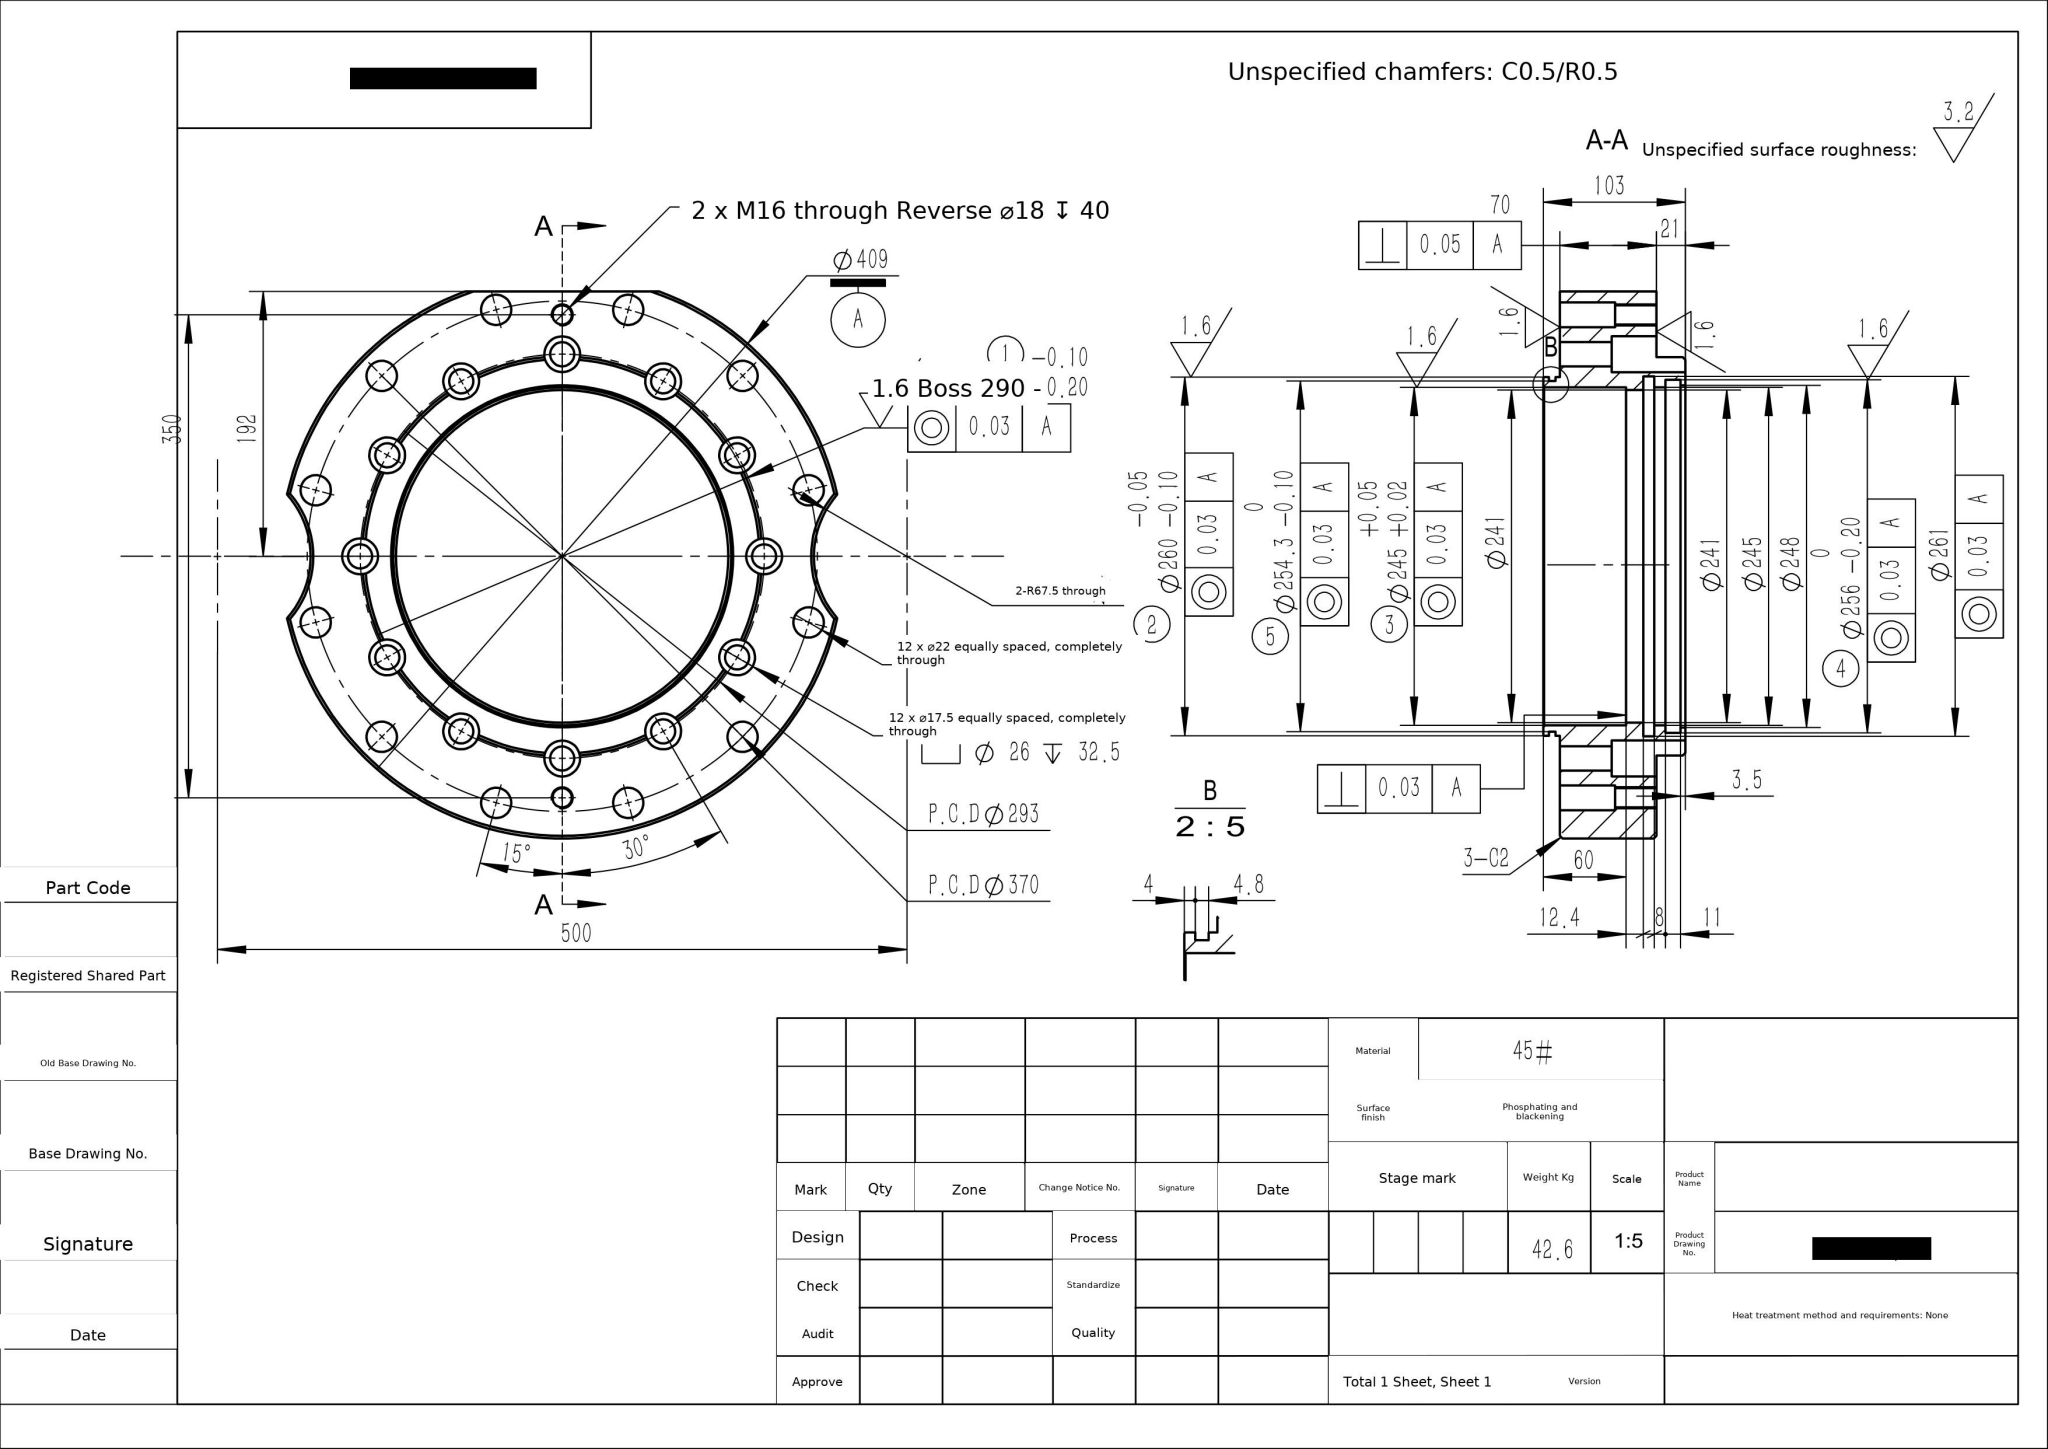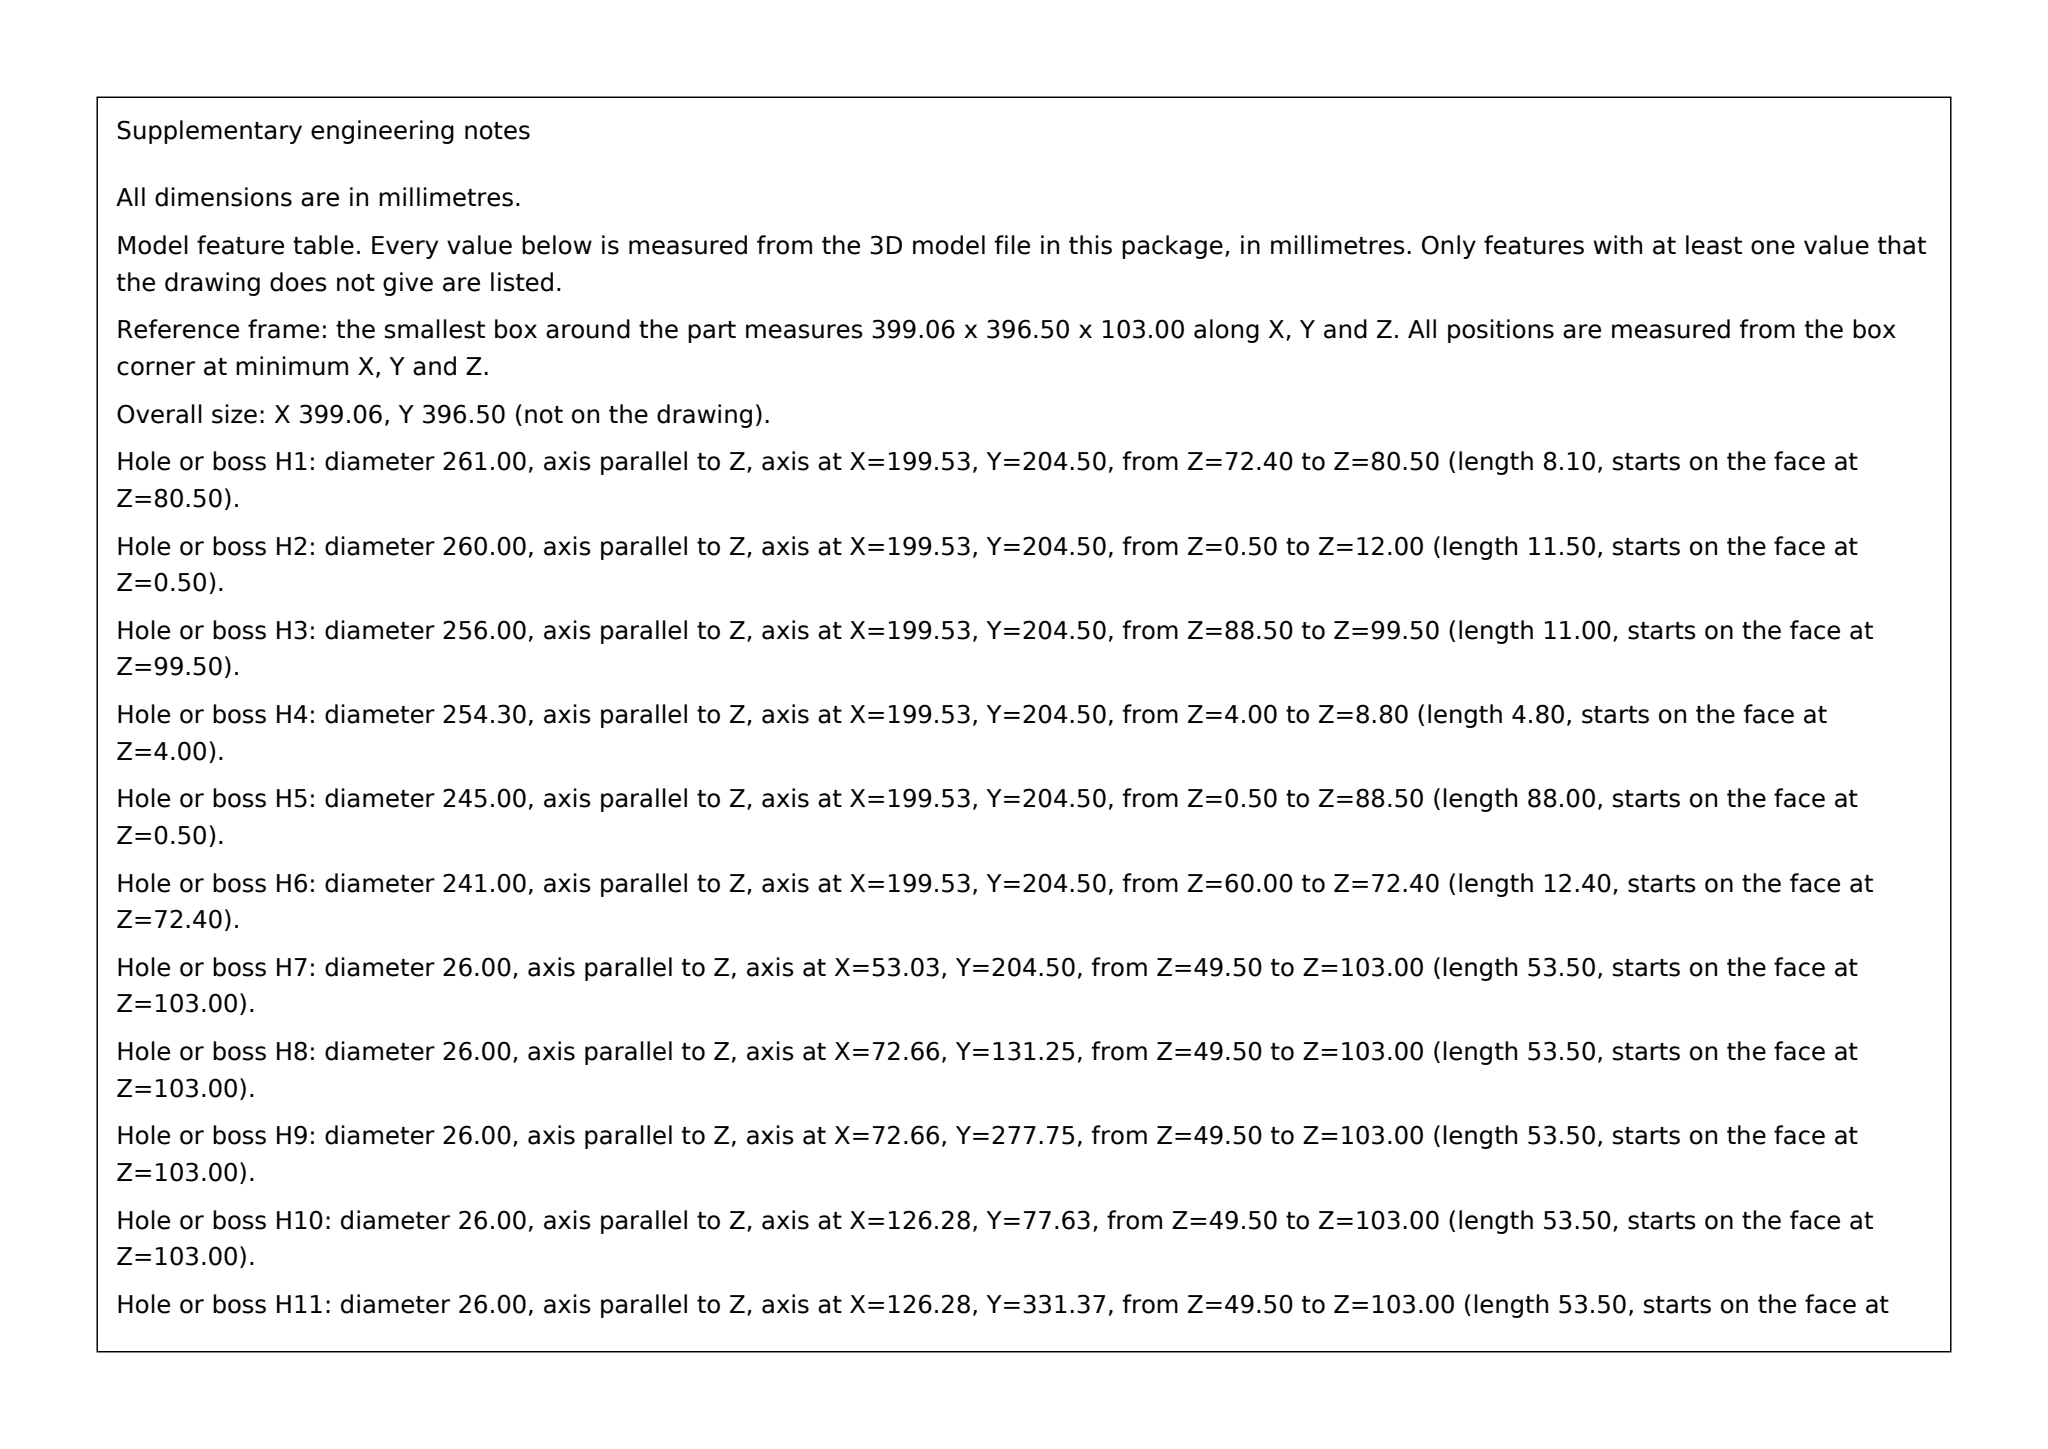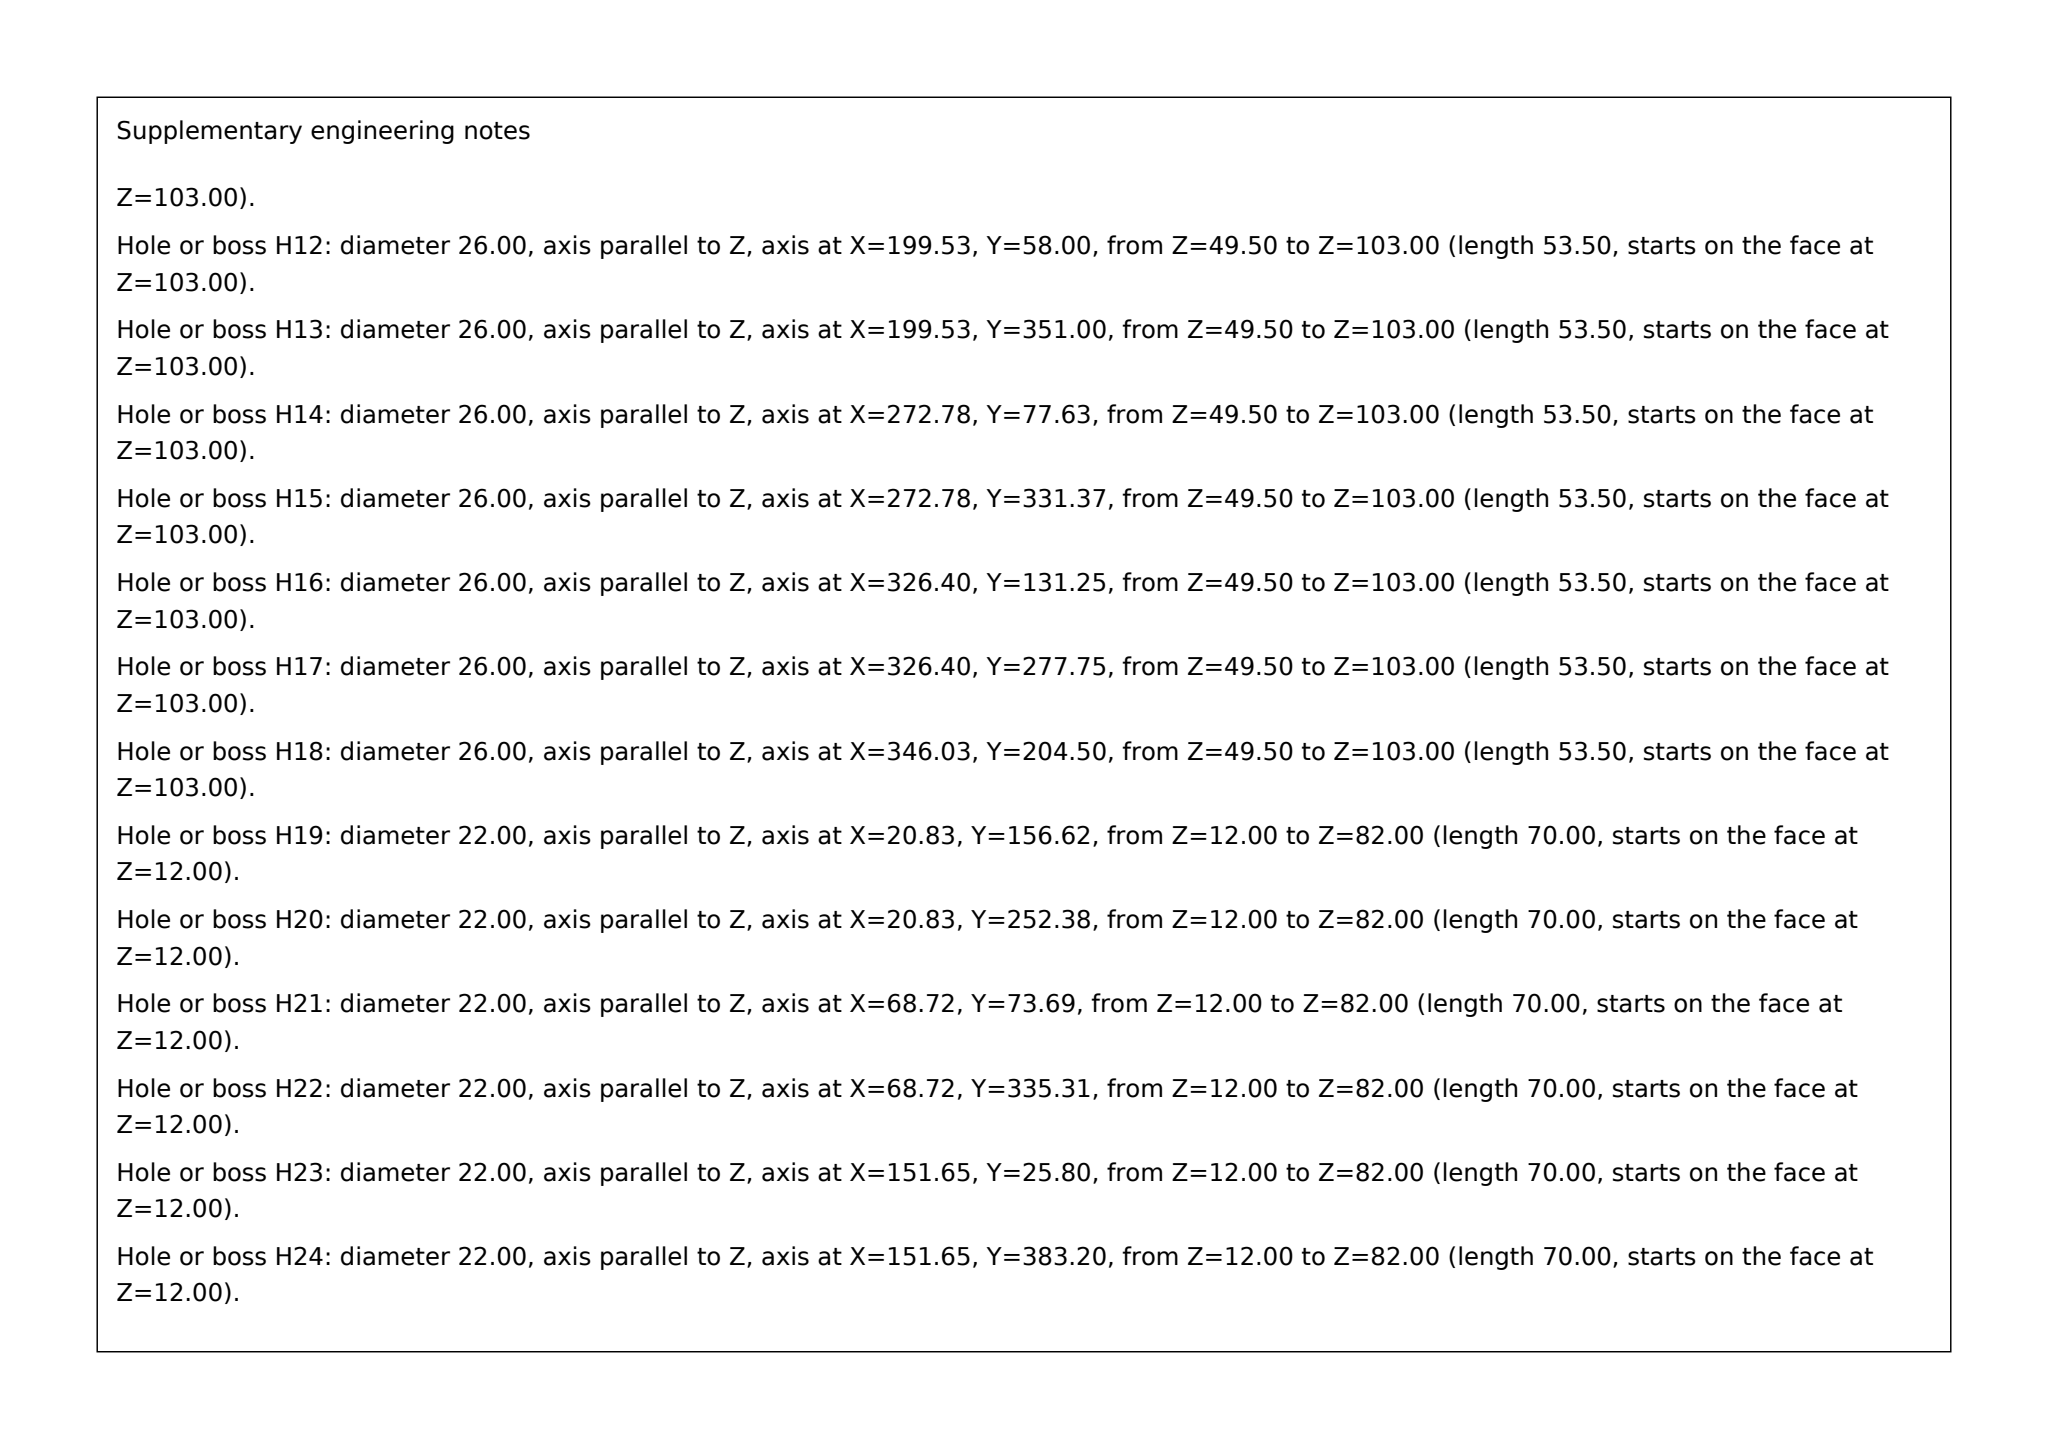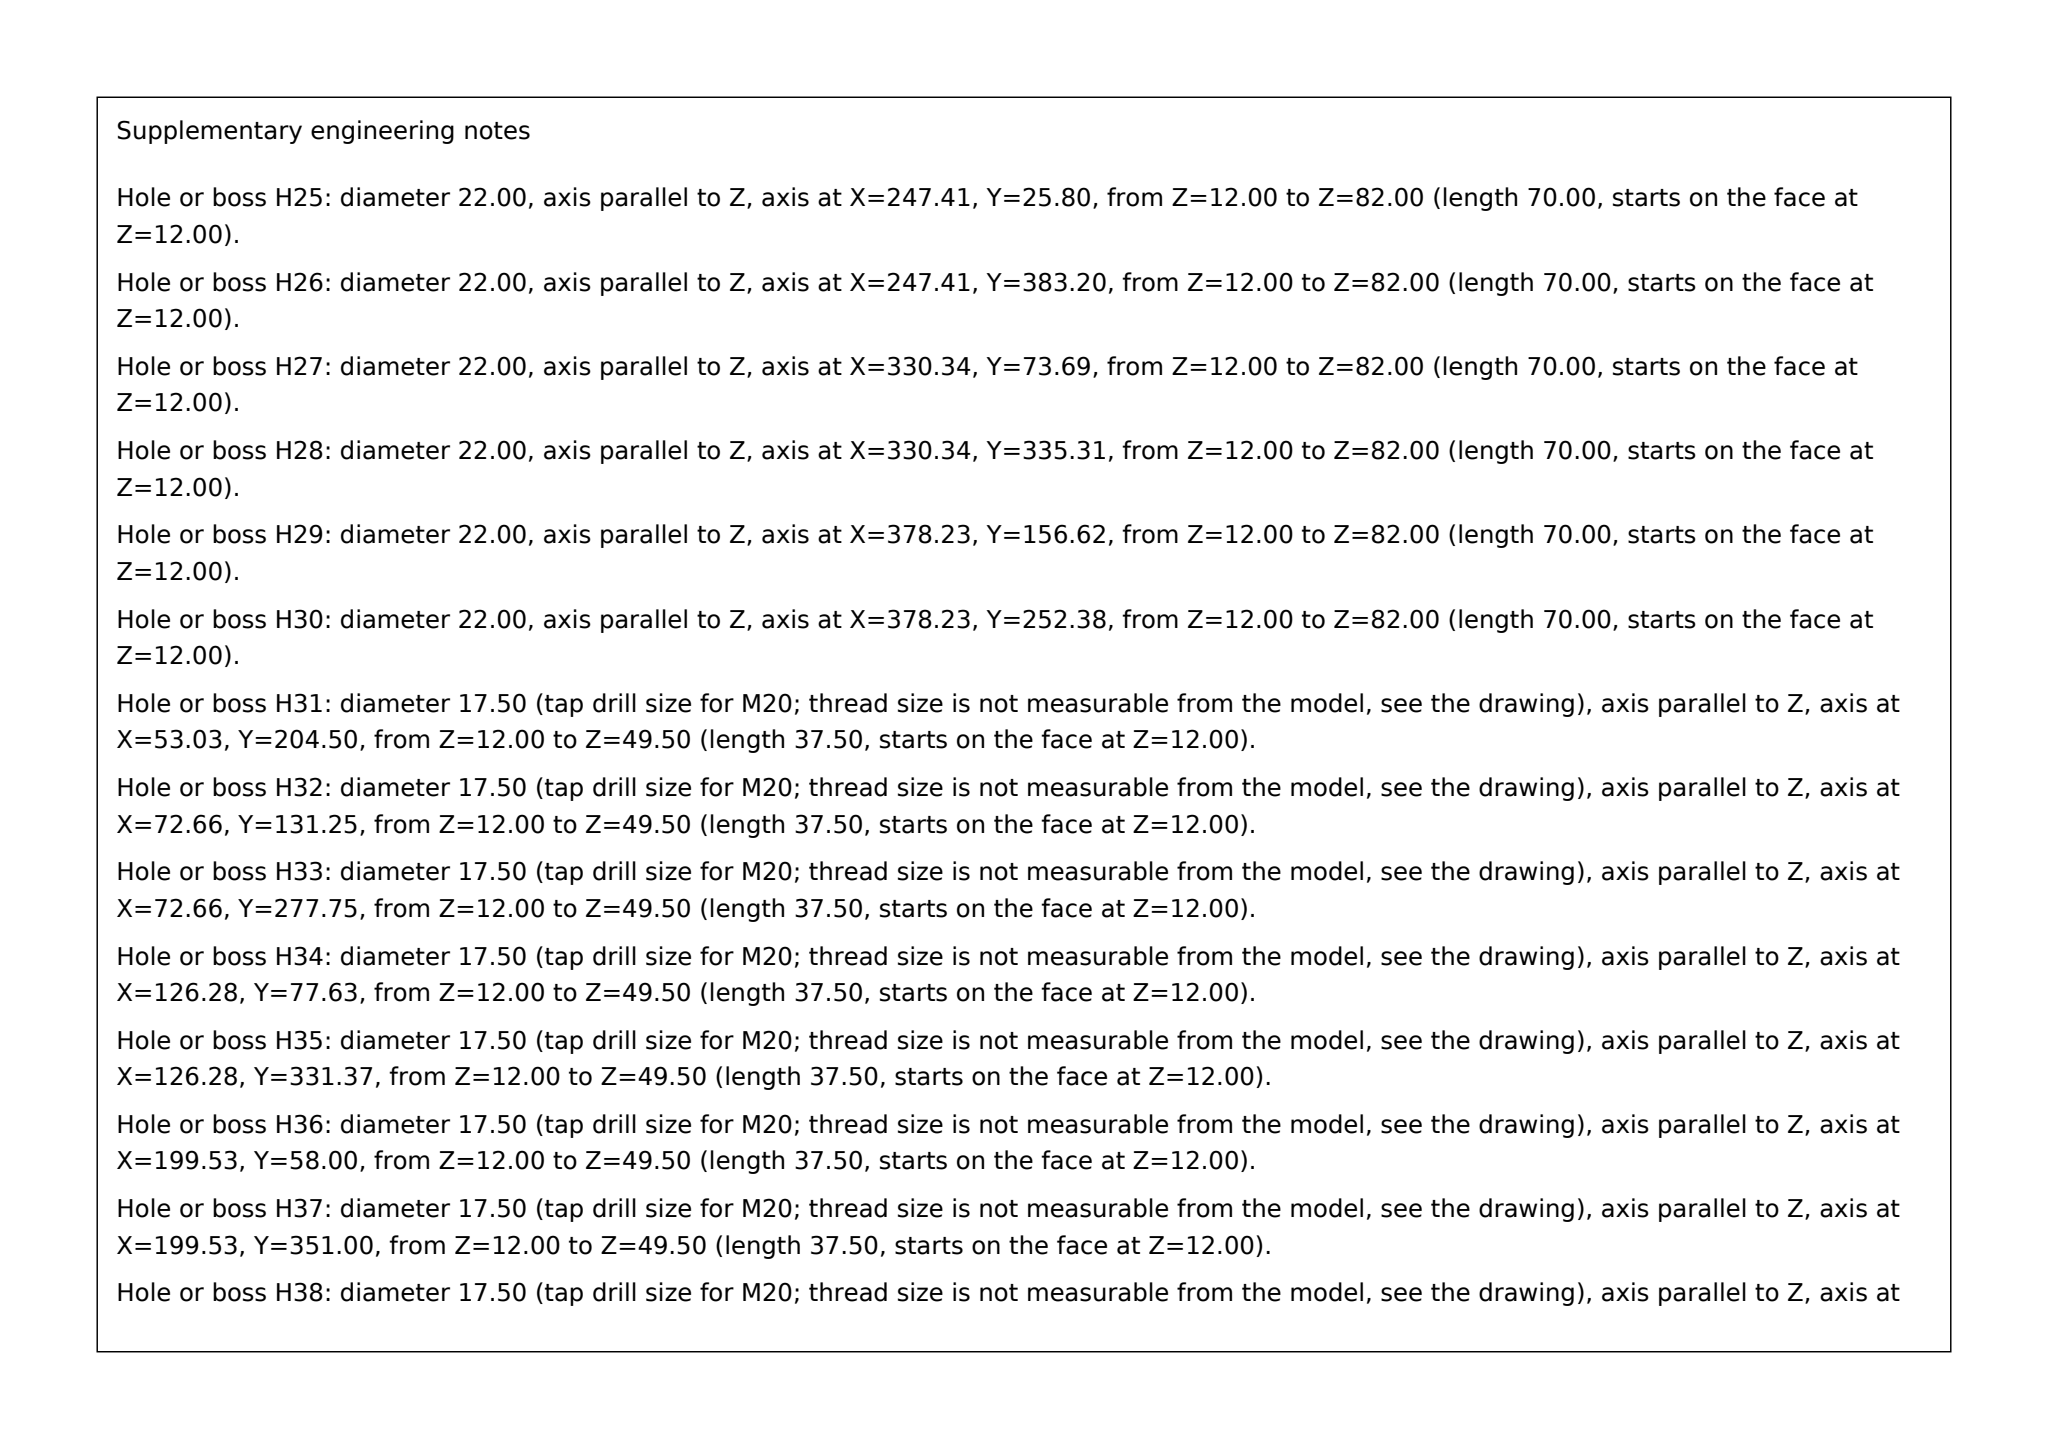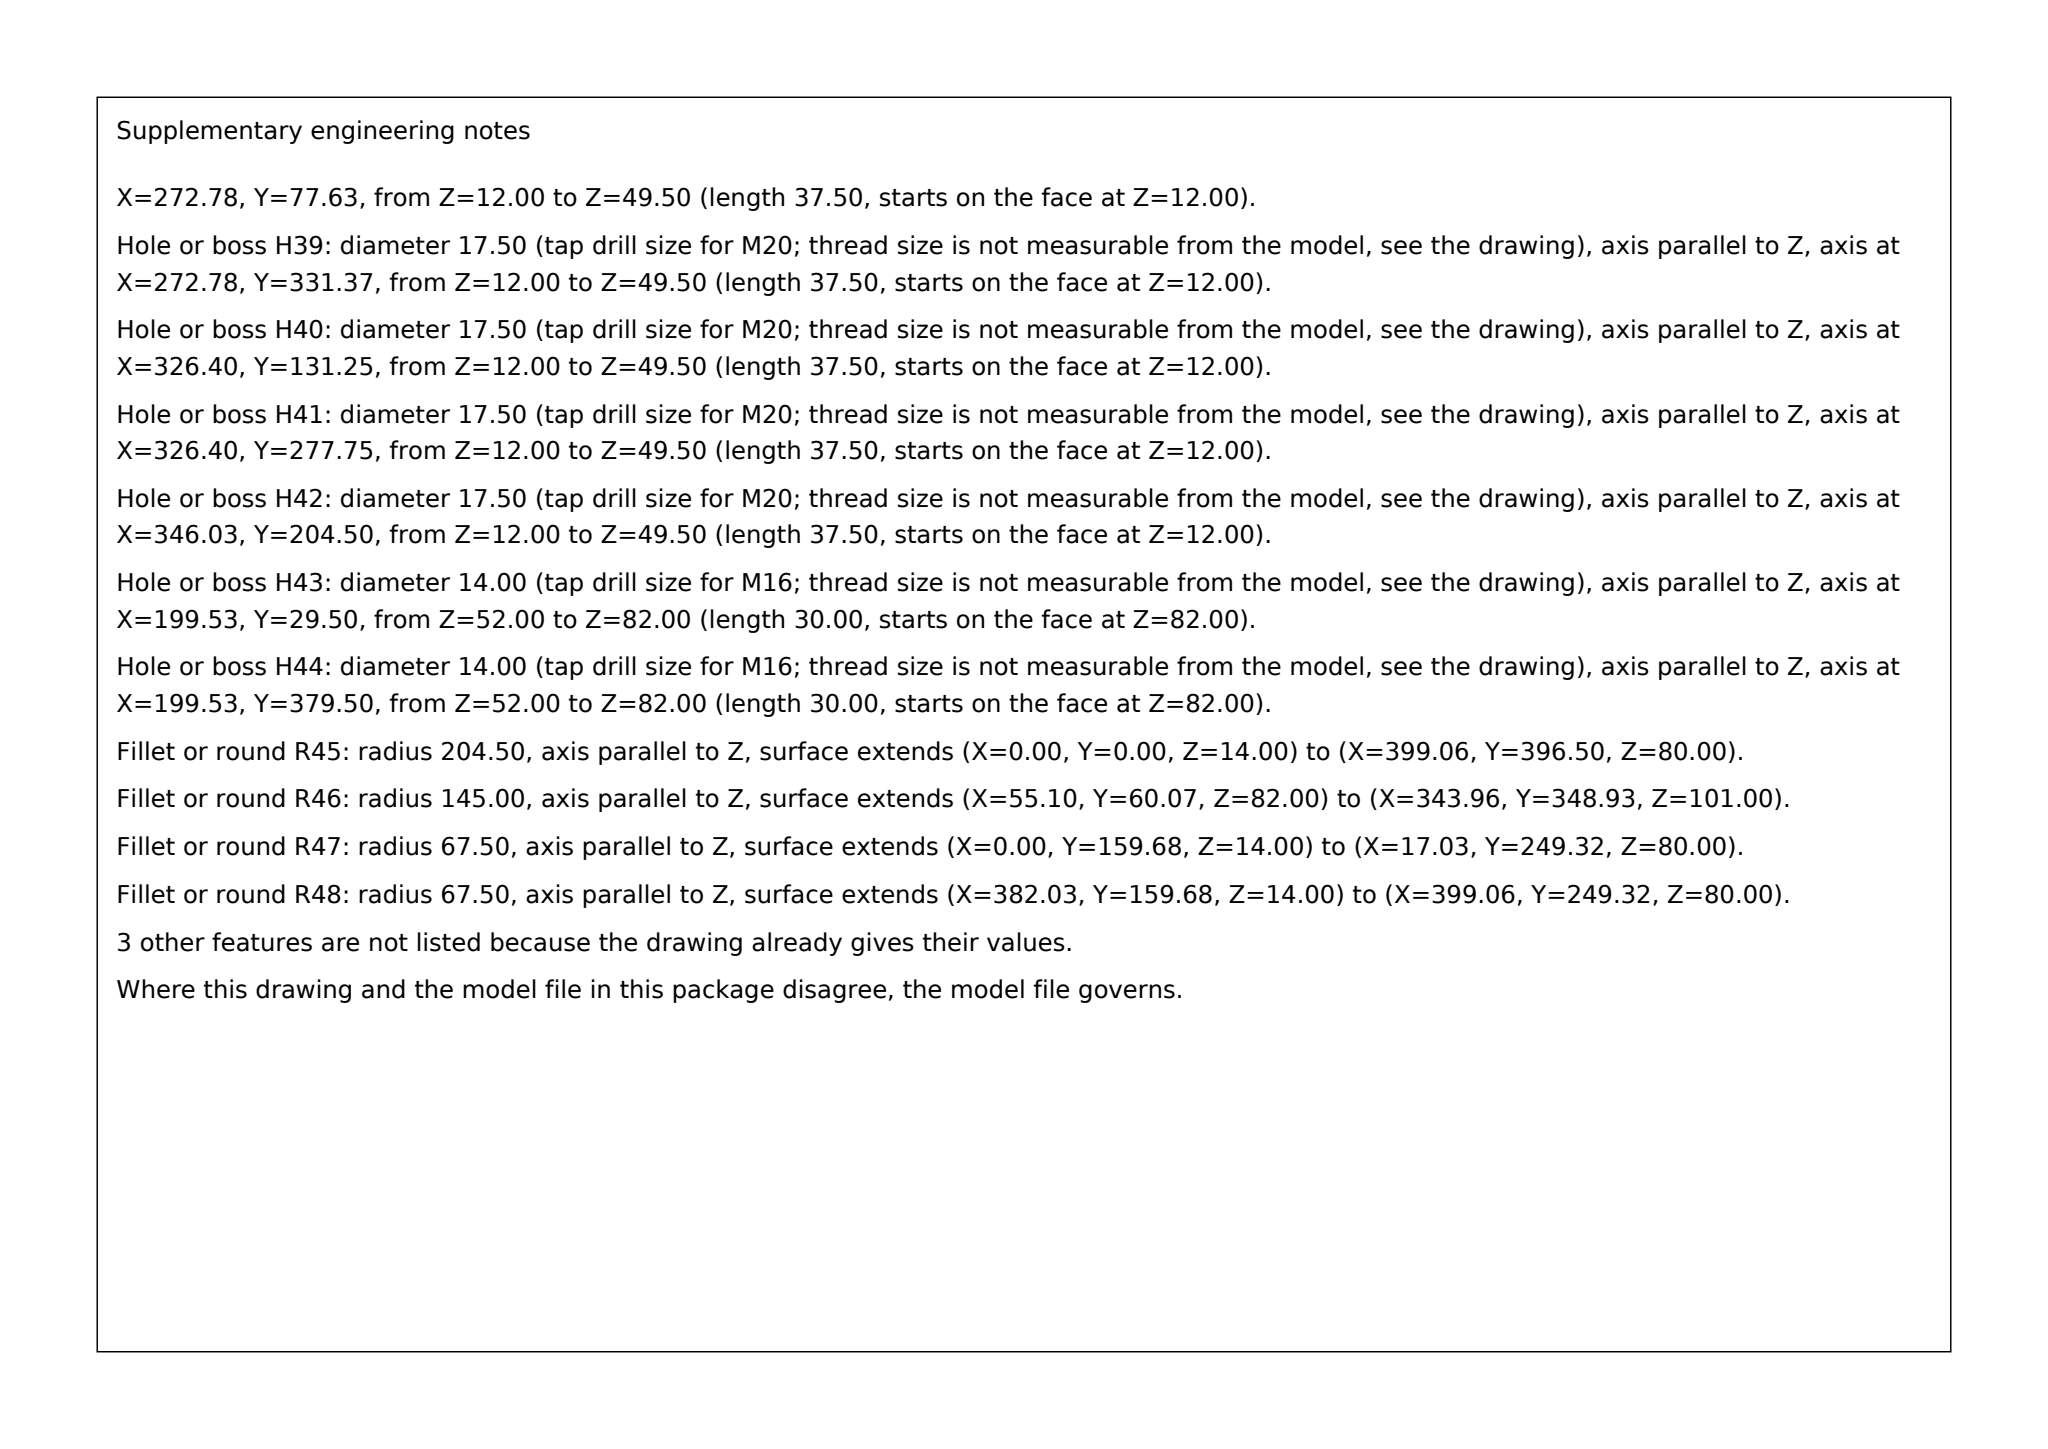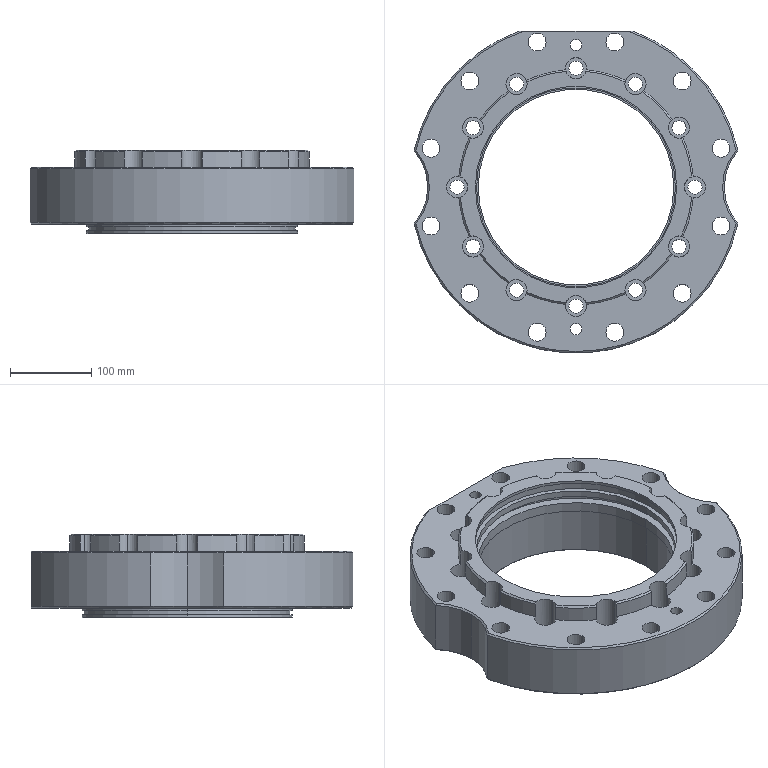Part | SolidWorks | mm | material 45# | 1 solid | 170 faces | box 399.06 x 396.5 x 103 mm | volume 5272947 mm3 | cylinder 116 | cone 28 | plane 26 | commonest cylinder face diameters 22 x24 26 x24 17.5 x24 290 x12 14 x4 18 x4 245 x4 260 x4
build123d program:
from build123d import *

# Parameters (mm, degrees)
SKETCH1_R              = 204.5
BOSS_EXTRUDE1_DEPTH    = 70
SKETCH2_R              = 130
BOSS_EXTRUDE2_DEPTH    = 12
BOSS_EXTRUDE3_START    = -63
SKETCH7_R              = 145
SKETCH7_R_2            = 65
BOSS_EXTRUDE3_DEPTH    = 35
CIRPATTERN1_COUNT      = 12
SKETCH13_R             = 75.5
CUT_EXTRUDE4_DEPTH     = 306.36
SKETCH14_R             = 77.5
CUT_EXTRUDE5_DEPTH     = 62
BOSS_EXTRUDE5_START    = -60
SKETCH15_R             = 204.5
SKETCH15_R_2           = 175
BOSS_EXTRUDE5_DEPTH    = 60
CHAMFER5_SIZE          = 3
CHAMFER5_SIZE2         = 1.092
CHAMFER7_SIZE          = 2
M20_CLEARANCE_HOLE_1_D = 22
CIRPATTERN3_COUNT      = 12
SKETCH29_R             = 120.5
CUT_EXTRUDE15_DEPTH    = 306.36
MOVE_FACE2_BY          = 5
CHAMFER10_SIZE         = 2
SKETCH30_R             = 13
CUT_EXTRUDE16_DEPTH    = 301.607
CIRPATTERN4_COUNT      = 12
CUT_EXTRUDE17_START    = -3.5
SKETCH31_R             = 128
CUT_EXTRUDE17_DEPTH    = 7
SKETCH32_R             = 124
CUT_EXTRUDE18_DEPTH    = 4
SKETCH33_R             = 122.5
CUT_EXTRUDE19_DEPTH    = 60
CUT_EXTRUDE20_START    = -12
SKETCH34_R             = 130.5
CUT_EXTRUDE20_DEPTH    = 8.1
CUT_EXTRUDE21_START    = -15
SKETCH35_R             = 122.5
CUT_EXTRUDE21_DEPTH    = 15
SKETCH36_R             = 128
CUT_EXTRUDE22_DEPTH    = 4
SKETCH37_W             = 200
SKETCH37_H             = 25
CUT_EXTRUDE23_DEPTH    = 301.607
CHAMFER11_SIZE         = 0.5
CUT_EXTRUDE24_START    = -4
SKETCH40_OUTSIDE_W     = 526.776
SKETCH40_OUTSIDE_H     = 514.276
SKETCH40_OUTSIDE_R     = 127.15
CUT_EXTRUDE24_DEPTH    = 4.8
SKETCH41_R             = 9
CUT_EXTRUDE25_DEPTH    = 40
M16_TAPPED_HOLE1_D     = 14
SKETCH44_R             = 67.5
CUT_EXTRUDE26_DEPTH    = 301.607
CHAMFER12_SIZE         = 2


with BuildPart() as part:
    # Sketch1 → Boss-Extrude1 (new body)
    with BuildSketch(Plane.XY):
        Circle(SKETCH1_R)
    extrude(amount=BOSS_EXTRUDE1_DEPTH)

    # Sketch2 → Boss-Extrude2 (add)
    with BuildSketch(Plane(origin=(0, 0, 0), x_dir=(-1, 0, 0), z_dir=(0, 0, -1))):
        Circle(SKETCH2_R)
    extrude(amount=BOSS_EXTRUDE2_DEPTH)

    # Sketch7 → Boss-Extrude3 (add)
    with BuildSketch(Plane(origin=(0, 0, -12), x_dir=(-1, 0, 0), z_dir=(0, 0, -1)).offset(BOSS_EXTRUDE3_START)):
        Circle(SKETCH7_R)
        Circle(SKETCH7_R_2, mode=Mode.SUBTRACT)
    extrude(amount=-BOSS_EXTRUDE3_DEPTH)

    # Sketch11 → Hole Size _ according to_ Hex Socket Hea (revolve, cut)
    with BuildSketch(Plane(origin=(0, 146.5, 70), x_dir=(0, -1, 0), z_dir=(1, 0, 0))):
        Polygon((0, 0), (0, 82), (8.75, 82), (8.75, 32.5), (13, 32.5), (13, 0), align=None)
    hole_size_according_to_hex_socket_hea = revolve(axis=Axis((0, 146.5, 76.35), (0, 0, -1)), mode=Mode.SUBTRACT)

    # CirPattern1: Hole Size _ according to_ Hex Socket Hea ×12 about axis
    cirpattern1_axis = Axis((0, 0, 0), (0, 0, 1))
    for i in range(1, CIRPATTERN1_COUNT):
        add(hole_size_according_to_hex_socket_hea.rotate(cirpattern1_axis, i * 360 / CIRPATTERN1_COUNT), mode=Mode.SUBTRACT)

    # Sketch13 → Cut-Extrude4 (cut, through all)
    with BuildSketch(Plane(origin=(0, 0, -12), x_dir=(-1, 0, 0), z_dir=(0, 0, -1))):
        Circle(SKETCH13_R)
    extrude(amount=-CUT_EXTRUDE4_DEPTH, mode=Mode.SUBTRACT)

    # Sketch14 → Cut-Extrude5 (cut)
    with BuildSketch(Plane(origin=(0, 0, -12), x_dir=(-1, 0, 0), z_dir=(0, 0, -1))):
        Circle(SKETCH14_R)
    extrude(amount=-CUT_EXTRUDE5_DEPTH, mode=Mode.SUBTRACT)

    # Sketch15 → Boss-Extrude5 (add)
    with BuildSketch(Plane.XY.offset(70).offset(BOSS_EXTRUDE5_START)):
        Circle(SKETCH15_R)
        Circle(SKETCH15_R_2, mode=Mode.SUBTRACT)
    extrude(amount=BOSS_EXTRUDE5_DEPTH)

    # Chamfer5
    chamfer5_edges = [part.edges().sort_by_distance(p)[0] for p in [
        (77.5, 0, -12),
    ]]
    chamfer5_side = [part.faces().sort_by_distance(p)[0] for p in [
        (77.5, 0, 19),
    ]]
    chamfer(chamfer5_edges, length=CHAMFER5_SIZE, length2=CHAMFER5_SIZE2, reference=chamfer5_side[0])

    # Chamfer7
    chamfer7_edges = [part.edges().sort_by_distance(p)[0] for p in [
        (-204.5, 0, 0),
        (-204.5, 0, 70),
    ]]
    chamfer(chamfer7_edges, length=CHAMFER7_SIZE)

    # M20 Clearance Hole 1 (through all)
    with Locations(Plane.XY.offset(70)):
        with Locations((-47.882, 178.696)):
            m20_clearance_hole_1 = Hole(M20_CLEARANCE_HOLE_1_D / 2)

    # CirPattern3: M20 Clearance Hole 1 ×12 about axis
    cirpattern3_axis = Axis((0, 0, 0), (0, 0, 1))
    for i in range(1, CIRPATTERN3_COUNT):
        add(m20_clearance_hole_1.rotate(cirpattern3_axis, i * 360 / CIRPATTERN3_COUNT), mode=Mode.SUBTRACT)

    # Sketch29 → Cut-Extrude15 (cut, through all)
    with BuildSketch(Plane.XY.offset(86)):
        Circle(SKETCH29_R)
    extrude(amount=-CUT_EXTRUDE15_DEPTH, mode=Mode.SUBTRACT)

    # Move Face2: a face moved outward by 5.0
    extrude(part.faces().sort_by_distance((72.5, -116, 86))[0], amount=MOVE_FACE2_BY, dir=(0, 0, 1))

    # Chamfer10
    chamfer10_edges = [part.edges().sort_by_distance(p)[0] for p in [
        (145, 0, 91),
    ]]
    chamfer(chamfer10_edges, length=CHAMFER10_SIZE)

    # Sketch30 → Cut-Extrude16 (cut, through all)
    with BuildSketch(Plane.XY.offset(70)):
        with Locations((0, 146.5)):
            Circle(SKETCH30_R)
    cut_extrude16 = extrude(amount=CUT_EXTRUDE16_DEPTH, mode=Mode.SUBTRACT)

    # CirPattern4: Cut-Extrude16 ×12 about axis
    cirpattern4_axis = Axis((0, 0, 91), (0, 0, -1))
    for i in range(1, CIRPATTERN4_COUNT):
        add(cut_extrude16.rotate(cirpattern4_axis, i * 360 / CIRPATTERN4_COUNT), mode=Mode.SUBTRACT)

    # Sketch31 → Cut-Extrude17 (cut)
    with BuildSketch(Plane.XY.offset(91).offset(CUT_EXTRUDE17_START)):
        Circle(SKETCH31_R)
    extrude(amount=-CUT_EXTRUDE17_DEPTH, mode=Mode.SUBTRACT)

    # Sketch32 → Cut-Extrude18 (cut)
    with BuildSketch(Plane.XY.offset(91)):
        Circle(SKETCH32_R)
    extrude(amount=-CUT_EXTRUDE18_DEPTH, mode=Mode.SUBTRACT)

    # Sketch33 → Cut-Extrude19 (cut)
    with BuildSketch(Plane(origin=(0, 0, -12), x_dir=(-1, 0, 0), z_dir=(0, 0, -1))):
        Circle(SKETCH33_R)
    extrude(amount=-CUT_EXTRUDE19_DEPTH, mode=Mode.SUBTRACT)

    # Sketch34 → Cut-Extrude20 (cut)
    with BuildSketch(Plane.XY.offset(80.5).offset(CUT_EXTRUDE20_START)):
        Circle(SKETCH34_R)
    extrude(amount=-CUT_EXTRUDE20_DEPTH, mode=Mode.SUBTRACT)

    # Sketch35 → Cut-Extrude21 (cut)
    with BuildSketch(Plane.XY.offset(80.5).offset(CUT_EXTRUDE21_START)):
        with Locations(Location((0, 0, 0), (0, 0, 180))):
            Circle(SKETCH35_R)
    extrude(amount=CUT_EXTRUDE21_DEPTH, mode=Mode.SUBTRACT)

    # Sketch36 → Cut-Extrude22 (cut)
    with BuildSketch(Plane.XY.offset(80.5)):
        Circle(SKETCH36_R)
    extrude(amount=-CUT_EXTRUDE22_DEPTH, mode=Mode.SUBTRACT)

    # Sketch37 → Cut-Extrude23 (cut, through all)
    with BuildSketch(Plane.XY.offset(70)):
        with Locations((0, 204.5)):
            Rectangle(SKETCH37_W, SKETCH37_H)
    extrude(amount=-CUT_EXTRUDE23_DEPTH, mode=Mode.SUBTRACT)

    # Chamfer11
    chamfer11_edges = [part.edges().sort_by_distance(p)[0] for p in [
        (122.5, 0, -12),
        (130, 0, -12),
    ]]
    chamfer(chamfer11_edges, length=CHAMFER11_SIZE)

    # Sketch40 outside → Cut-Extrude24 (cut)
    with BuildSketch(Plane(origin=(0, 0, -12), x_dir=(-1, 0, 0), z_dir=(0, 0, -1)).offset(CUT_EXTRUDE24_START)):
        with Locations((0, -6.25)):
            Rectangle(SKETCH40_OUTSIDE_W, SKETCH40_OUTSIDE_H)
        Circle(SKETCH40_OUTSIDE_R, mode=Mode.SUBTRACT)
    extrude(amount=-CUT_EXTRUDE24_DEPTH, mode=Mode.SUBTRACT)

    # Sketch41 → Cut-Extrude25 (cut)
    with BuildSketch(Plane(origin=(0, 0, 0), x_dir=(-1, 0, 0), z_dir=(0, 0, -1))):
        with Locations((0, 175)):
            Circle(SKETCH41_R)
        with Locations((0, -175)):
            Circle(SKETCH41_R)
    extrude(amount=-CUT_EXTRUDE25_DEPTH, mode=Mode.SUBTRACT)

    # M16 Tapped Hole1 (through all)
    with Locations(Plane(origin=(0, 0, 40), x_dir=(-1, 0, 0), z_dir=(0, 0, -1))):
        with Locations((0, -175), (0, 175)):
            Hole(M16_TAPPED_HOLE1_D / 2)

    # Sketch44 → Cut-Extrude26 (cut, through all)
    with BuildSketch(Plane.XY.offset(70)):
        with Locations((-250, 0)):
            Circle(SKETCH44_R)
        with Locations((250, 0)):
            Circle(SKETCH44_R)
    extrude(amount=-CUT_EXTRUDE26_DEPTH, mode=Mode.SUBTRACT)

    # Chamfer12
    chamfer12_edges = [part.edges().sort_by_distance(p)[0] for p in [
        (182.5, 0, 0),
        (182.5, 0, 70),
        (-182.5, 0, 0),
        (-182.5, 0, 70),
    ]]
    chamfer(chamfer12_edges, length=CHAMFER12_SIZE)


solid = part.part